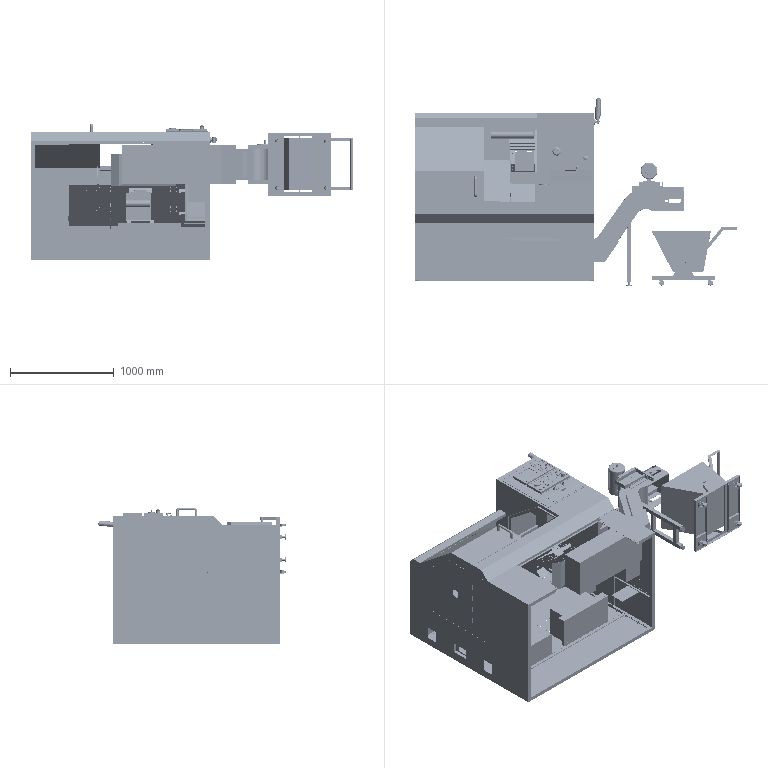Assembly | SolidWorks | mm | 112 component files | 213 solids | 6594 faces | box 3103.3 x 1799.75 x 1316.5 mm | volume 83821011 mm3 | plane 4108 | cylinder 2360 | cone 62 | torus 44 | sphere 16 | spline 4 | commonest cylinder face diameters 3 x356 4 x356 7 x259 6 x244 10 x225 5.2 x144 14 x52 8 x48
Bill of materials:
GuardWheel | 4 |  | L-shaped (right-angle) plate body carrying a long cylinder and a shorter cylinder, with slotted fork-like flat tabs at the cylinder ends.
Telescopic | 1 |  | Bent thin-sheet bracket with stepped/notched outline: a large flat panel, an offset narrower flange, and a downturned flange with an irregular notched edge.
Baffle | 1 |  | Thin flat U-shaped (inverted-U) plate with a large rectangular open cutout and many small through-holes, plus a downturned flange along one edge.
BaffleFixingBracket | 1 |  | Slender bent-strap bracket in a Z/offset shape, with U-channel style ends that each carry flat tabs with small holes.
Bracket | 2 |  | Long straight channel/angle strip formed as a folded right-angle (V-shaped) section, with two small holes along its length.
Cart | 1 |  | Open hopper/bin-like box with a trapezoidal (tapered) side profile, short pin stubs on opposite sides, and a bent rod-style handle loop sticking out of one side.
ChipCollectorCartChassis | 1 |  | Rectangular frame plate with a large central rectangular opening, side channel walls, and a tapered central tab ending in a small ring/eyelet.
TY-07-02-00BlackSmallRubberWheel | 4 |  | Caster-like wheel unit: square mounting plate with four corner holes, a fork/yoke bracket, and a single rounded cylindrical wheel on an axle.
Casing | 1 |  | Large sheet-metal style frame/enclosure with rectangular windows, a chamfered corner, folded side walls, and an attached long cantilever channel arm.
ChipConveyor1 | 1 |  | Elongated inclined channel/chute-like structure: a long box section that steps up through a curved incline to a raised head section with a plate and slots, held by a rod frame with a leg and knob-ended rods.
ControlBox | 1 |  | Shallow rectangular box/tray frame with a chamfered lower edge, two rectangular openings in the top, recessed side pockets, and round holes in the end walls.
ControlBoxDoor | 1 |  | Thin rectangular flat panel/lid with a rounded-corner rectangular slot (hand-hole like) and short pin stubs at both ends of one edge; a rolled or rounded lobe is seen along that edge.
ControlBoxRearPanel | 1 |  | Thin flat square plate with one small round through-hole near each of the four corners.
CopyOfSystem | 1 |  | Rectangular panel-style body made of a shallow top housing over a thin perimeter flange with mounting holes and a deeper, narrower rectangular box underneath. The top face has a raised rim border, a grid of small square key-like pads, a large round recess with a cylindrical boss inside it, a short pin, several low round buttons, a domed cylindrical knob, and a small rectangular block.
System | 1 |  | Rectangular housing with a flanged top. A thin perimeter flange with mounting holes sits on top of a deep rectangular box. The top surface is split into two raised sections: a larger one with a shallow rectangular recess and a row of small tabs along one edge, and a smaller one with a recessed field holding a grid of small square pads.
1_1 | 1 |  | Stepped cylindrical part: a larger-diameter head with a smaller-diameter shank below it. The head has a slot or partial cut-away, a cylindrical cross pin running through the slot, and the pin ends stick out slightly on both sides of the head. The shank has a chamfered end.
2_1 | 1 |  | Round bar or tube bent into a U shape, with two parallel legs joined by a long straight span through rounded bends. Each leg end has a small cross hole.
3_1 | 1 |  | Hexagonal nut-shaped body with a central round bore and chamfered corners on both faces.
4_1 | 1 |  | Plain flat annular washer-shaped ring: a circular disk with a concentric central hole and uniform thickness.
5_1 | 1 |  | Stepped cylindrical part: a larger-diameter head with a smaller-diameter shank below it. The head has a slot or partial cut-away, a cylindrical cross pin running through the slot, and the pin ends stick out slightly on both sides of the head. The shank has a chamfered end.
6 | 1 |  | Hexagonal nut-shaped body with a central round bore and chamfered corners.
7_1 | 1 |  | Plain flat annular washer-shaped ring: a circular disk with a concentric central hole and uniform thickness.
ControlBoxGasket | 2 |  | Very thin flat annular ring (shim-like): a circular disk with a large concentric central hole.
ControllerRotatingShaft | 2 |  | Flanged sleeve: a thin-walled cylindrical tube with a thin flat circular flange at one end, and four evenly spaced round through-holes in the flange.
Door | 1 | Plain Carbon Steel | Sheet panel bent into a profile with three sections: horizontal, sloped, and vertical. A large rounded-rectangle window is cut through the sloped section, and the panel has small holes and slots.
DoorGlass | 1 |  | Thin flat rectangular plate set at an incline, with no visible holes or features.
ElectricalBoxCoverPlate | 1 |  | Long, narrow, flat rectangular strip with small holes at both ends and at mid-length.
ElectricalBoxCoverPlate2 | 1 |  | Flat rectangular strip, shorter and wider in proportion than a long bar, with six small holes: four at the corners and two at mid-length.
FixedBracket2 | 1 |  | Bent sheet bracket with an L-shaped (angle) cross-section. One leg tapers along its length, and the other leg has two round holes.
FixedFrame | 1 |  | Bent sheet angle bracket similar to a tapered L-bracket, with two round holes in one leg and a tapered opposite leg; it appears to be mirrored or oriented differently from the similar part.
FrontBaffle | 1 |  | Sheet panel bent into a horizontal, sloped, and vertical section profile, with no large window, and with a row of small holes along the bent edges.
FrontReceivingPlate | 1 |  | Long bent angle strip with two legs at a non-right (acute) angle and tapered or angled cut ends.
FuelTank | 1 |  | Rectangular box-shaped body with a flange plate at one face that extends slightly beyond the box outline, with four corner holes. One hole is also visible on the top face.
FuelTankCap | 1 |  | Flat thin rectangular plate with four round holes near the corners.
1 | 1 |  | Complex multi-bend sheet bracket with several panels, side legs, notches, stepped tabs, and an offset cutout region.
2 | 1 |  | Bent sheet part with a broad, channel-like body, two side legs, a central opening between two sloped panels, and a small central tab with a hole.
3 | 1 |  | Thin bent sheet-metal panel: a large flat plate with a wide rectangular cutout that leaves two parallel legs, plus a narrow bent strip/flange along the solid edge carrying small holes; the side view shows the main plate inclined at roughly 45 degrees and a short stepped (Z-like) flange at one end.
TieRod1 | 4 |  | Flat bar link with fully rounded ends and one round through-hole near each end.
TieRod2 | 2 |  | Long, slender flat bar with rounded ends and three small through-holes, one at each end and one at mid-length.
GlassPressFrame | 1 |  | Thin flat rectangular frame or gasket-like plate with a large central rectangular opening and eight small holes around the border (four corners and four edge midpoints).
Handle | 1 |  | U-shaped bent round rod: one straight crossbar joined to two parallel straight legs by radiused bends, with the legs ending in flat cut faces.
IlluminationLamp | 1 |  | Elongated half-round (D-section) body with a flat back face and a curved front, closed at each end by a plate that projects past the flat side and has two small notches on its edge.
LampHolder | 1 |  | Sheet-metal hat-section channel: a web, two parallel side walls and outward-turned flanges along both free edges, with two small holes near each end of the web.
Base | 1 |  | Flanged bushing-like part: a circular flange disc with three through-holes, and a short, slightly tapered cylindrical hub with a central through-bore.
LED | 1 |  | Elongated cylindrical housing with a rounded closed end. The other end has a smaller stepped spigot with a bore, surrounded by a ring of small holes/pockets on the end face. There is a circular patch of parallel slots on the side near the spigot end, and faint circumferential seam lines along the body.
RotatingHead | 1 |  | Cylindrical disc/eye body with a central through-hole, plus a two-diameter stepped cylindrical pin projecting radially from its side; the underside face shows a small hole and an arc-shaped groove.
UpperRotatingHead | 1 |  | Cylindrical disc/eye body with a chamfered central through-bore, plus a two-diameter stepped cylindrical pin projecting radially from its side; the outer edges and pin end are chamfered.
LeftGuardBracket | 2 |  | Long sheet-metal angle bracket: an L-section strip with two round holes in one leg, plus a perpendicular bent end tab with a single round hole.
LeftLowerSkirt | 1 |  | L-shaped bent sheet: a long rectangular leg and a shorter perpendicular leg joined at one bend.
LeftMaterialInletPlate | 1 |  | Thin plate with a single obtuse bend, giving two flat panels at an angle.
LeftSideGuardPlate | 1 |  | Thin flat rectangular strip or plate with no visible holes.
LeftWindow | 1 |  | Flat panel with one chamfered (angled) corner, a large round hole, a grid of parallel slots, and small holes around the edge.
LowerBaffle | 1 |  | Thin flat plate with a stepped, chamfered upper outline and a rounded notch at one lower corner.
LowerRightPlateBracket | 1 |  | L-shaped bracket: a wide flat flange and a short perpendicular flange, each with two round holes.
LowerRightSurroundCoverPlate | 1 |  | Thin flat rectangular plate with one small round hole near each of the four corners.
MiddleBaffle | 1 |  | Flat polygonal plate with angled edges and stepped tabs, a large central circular opening, and many small holes.
Motor | 1 |  | Cylindrical body with lengthwise ribs, a small protruding shaft on one end, a rounded dome on the other end, a rectangular box on one side, and a flat foot base.
OilTankBracket | 1 |  | Wedge-shaped (tapered) solid block with small holes on two faces.
Axis | 2 |  | Flanged cylindrical bushing with a through-bore and a shallow ring-shaped groove near the top end.
Bearing | 2 |  | Short annular ring (washer- or bearing-like shape) with a central bore and concentric ring grooves on one face.
Pulley | 2 |  | Short ring with a through-bore and a groove around the outside, which gives it a spool-like profile of two thin outer flanges joined by a smaller-diameter hub.
RearBaffle | 1 |  | Thin rectangular plate with a low raised rim around its edge, like a shallow tray. It has twelve groups of short parallel slots and small pins or holes along two opposite edges.
RearCoverPlate | 1 |  | Long, shallow, open-faced rectangular pan or channel: a flat web with walls on all four edges. The walls have small holes.
RearFixingPlate | 1 |  | Thin, flat rectangular plate with four round through-holes in a rectangular pattern near the corners.
RearLowerSkirt | 1 |  | Long angle-shaped piece: a long flat base with a short upright wall at one end. It has a few small holes and a fine line or groove along one long edge.
RightSideBaffle | 1 |  | Rectangular block or bar with a step (notch) at one end. It is set at an angle to the view axes.
RightSideLowerBaffle | 1 |  | Bent sheet-metal panel: a tall flat main panel with a large stepped rectangular window cut out, and a 90-degree flange along the top. The flange has slotted holes and a stepped (notched) outline.
RightSideWindow | 1 |  | Very thin flat plate shaped like a five-sided polygon: a near-square with one corner cut off at about 45 degrees. It has small holes near the edges.
Telescopic1 | 1 |  | Bent sheet-metal bracket. In profile it has a sloped leg at about 45 degrees running into a horizontal leg that ends in a short turned-down lip. The sloped leg has stepped tabs, and the plan view shows a rectangular notch cut from one side.
Telescopic2 | 1 |  | Bent sheet-metal bracket with a profile similar to the previous bracket: a sloped leg into a horizontal leg ending in a short lip, with stepped tabs on the sloped leg. The plan view is a plain rectangle with no notch.
Telescopic3 | 1 |  | Bent bracket with a sloped leg joined to a horizontal leg. The sloped leg has two raised strips or tabs, each carrying a pair of small holes.
WheelAssembly | 4 |  | Compact L-shaped (90-degree) body with rectangular pockets that hold two cylinders of different lengths. Both cylinders have axial holes. There are forked (slotted) end tabs.
RoundBaffle | 1 |  | Thin flat ring (annulus) with four small through-holes spaced evenly around the rim.
ScraperPlate | 1 |  | Thin flat strip in a joggled/Z shape in plan: a straight end section, a diagonal middle section and a second straight end section, with a single row of small holes along the centerline.
Section1 | 1 |  | Formed sheet-metal channel or cover: a rectangular main panel with folded side walls, end walls with a stepped central notch along the bottom edge, and a small tab with a hole at one corner.
Section2 | 1 |  | Formed sheet-metal channel or cover: a rectangular panel with folded side and end walls, and end walls with a stepped notch along the bottom edge that has angled corners. Very similar to the other channel parts, but it has no corner tab hole.
Section3 | 1 |  | Formed sheet-metal channel or cover with folded walls and a stepped bottom-edge notch in the end walls. Its proportions are a little longer and narrower than the other channel variants.
Section4 | 1 |  | Formed sheet-metal channel or cover, the narrowest and most elongated of the similar variants, with folded walls and a stepped notch along the bottom edge in the end walls.
Section5 | 1 |  | Formed sheet-metal bracket: a central channel section with rectangular openings, and two angled mounting legs that each carry four elongated slots and have rounded corners.
SlideRail | 1 |  | Long, thin, flat bar with four evenly spaced small holes along its centerline.
ElectricalBoxDoor | 1 |  | Thin flat rectangular plate with one small elongated slot near one long edge. The slot has narrow extensions at each end.
ElectricalBoxTopPlate | 1 |  | Thin flat rectangular plate with one small round hole near each of its four corners.
TransformerBox | 1 |  | Rectangular box-shaped sheet-metal enclosure. It has small holes along its edges, two small rectangular cutouts in one long side wall, a rectangular patch or recess on the top face, and inturned flanges or a lip around one open or edge side.
TransformerBoxPlate | 1 |  | Flat rectangular plate with a large central rectangular opening and four round holes near the corners.
UpperSlideBearing | 2 |  | Short annular ring (thick washer/ring shape) with a central through-bore; one face shows concentric inner and outer rings separated by a recessed annular groove.
UpperSlideFixedBlock | 2 |  | Solid stepped cylinder: a large-diameter disc-like section with a smaller coaxial cylindrical boss projecting from one face.
UpperBaffle | 1 |  | Long straight prismatic profile of constant cross-section; the section is a bent bar with a short flat leg, an angled transition segment, and a longer perpendicular leg (a joggled/offset angle shape).
UpperCoverBracket2 | 1 |  | Thin-walled sheet-style bracket: two triangular side plates, each with a tapered lightening cutout with rounded corners, joined by a rectangular web with a large central opening and bent flanges carrying round holes.
UpperGuardBracket | 1 |  | Thin-walled sheet-style bracket similar to a U-shaped frame: two triangular side plates with large tapered rounded-corner lightening cutouts, joined by a crossbar, with leg flanges carrying elongated slots and round holes.
WaterPump | 1 |  | Compound cylindrical assembly-like body: a large cylinder with a rectangular block underneath, a thin square flange plate with four corner holes, and parallel rods plus a flat bar extending to a cylindrical end disc.
Mates:
1. coincident | Casing-1 face at (-858.301, 497.073, 511.481) dir (0, 0, 1) | Door-1 face at (-869.55, -18.434, 511.481) dir (0, 0, 1)
2. distance | Door-1 face at (-869.55, -314.434, 481.481) dir (0, -1, 0) | Casing-1 face at (-869.55, -318.434, 129.481) dir (0, 1, 0)
3. coincident | Casing-1 face at (-871.55, -30.485, 476.481) dir (0, 0, -1) | FrontBaffle-1 face at (-294.55, -318.432, 476.481) dir (0, 0, 1)
4. coincident | Casing-1 face at (-871.55, 371.566, 162.364) dir (0, -1, 0) | FrontBaffle-1 face at (-294.55, 371.566, 162.363) dir (0, 1, 0)
5. distance | FrontBaffle-1 face at (-294.55, -36.686, 386.009) dir (1, 0, 0) | Casing-1 face at (-869.55, 406.571, 129.481) dir (1, 0, 0)
6. coincident | Casing-1 face at (240.45, 497.073, -448.519) dir (-1, 0, 0) | UpperBaffle-1 face at (240.45, 486.18, 119.594) dir (1, 0, 0)
7. coincident | Casing-1 face at (-934.55, 541.566, 511.481) dir (0, 1, 0) | UpperBaffle-1 face at (240.45, 541.566, 136.486) dir (0, 1, 0)
8. concentric | Door-1 face at (-354.55, -345.434, 473.481) dir (0, 0, 1) r 3.5 | PulleyAssembly-1/Axis-1 face at (-354.55, -345.434, 482.181) dir (0, 0, 1) r 1.65
9. coincident | Door-1 face at (-269.55, -538.432, 483.481) dir (0, 0, 1) | PulleyAssembly-1/Axis-1 face at (-354.55, -345.434, 483.481) dir (0, 0, -1)
10. concentric | Door-1 face at (-754.55, -345.434, 473.481) dir (0, 0, 1) r 3.5 | PulleyAssembly-2/Axis-1 face at (-754.55, -345.434, 482.181) dir (0, 0, 1) r 1.65
11. coincident | Door-1 face at (-269.55, -538.432, 483.481) dir (0, 0, 1) | PulleyAssembly-2/Axis-1 face at (-754.55, -345.434, 483.481) dir (0, 0, -1)
12. coincident | Casing-1 face at (-858.301, 497.073, 491.481) dir (0, 0, -1) | SlideRail-1 face at (-791.2, -396.75, 491.481) dir (0, 0, 1)
13. distance | SlideRail-1 face at (235.45, -361.434, 491.481) dir (1, 0, 0) | Casing-1 face at (240.45, 497.073, -448.519) dir (-1, 0, 0)
14. tangent | PulleyAssembly-1/Pulley-1 face at (-354.55, -345.434, 494.431) dir (0, 0, 1) r 16 | SlideRail-1 face at (-897.55, -361.434, 491.481) dir (0, 1, 0)
15. tangent | PulleyAssembly-2/Pulley-1 face at (-754.55, -345.434, 494.431) dir (0, 0, 1) r 16 | SlideRail-1 face at (-897.55, -361.434, 491.481) dir (0, 1, 0)
16. coincident | Door-1 face at (-911.609, 394.568, -8.567) dir (0, -1, 0) | UpperAxis-1/UpperSlideFixedBlock-1 face at (-778.65, 394.568, -31.569) dir (0, 1, 0)
17. tangent | Door-1 face at (-776.05, 386.568, -35.567) dir (-1, 0, 0) | UpperAxis-1/UpperSlideFixedBlock-1 face at (-778.65, 386.568, -31.569) dir (0, 1, 0) r 2.6
18. tangent | Casing-1 face at (-858.301, 497.073, -17.569) dir (0, 0, -1) | UpperAxis-1/UpperSlideBearing-1 face at (-778.65, 382.968, -31.569) dir (0, 1, 0) r 14
19. coincident | Door-1 face at (-911.609, 394.568, -8.567) dir (0, -1, 0) | UpperAxis-2/UpperSlideFixedBlock-1 face at (-323.45, 394.568, -31.569) dir (0, 1, 0)
20. tangent | Door-1 face at (-326.05, 386.568, -35.567) dir (-1, 0, 0) | UpperAxis-2/UpperSlideFixedBlock-1 face at (-323.45, 386.568, -31.569) dir (0, 1, 0) r 2.6
21. tangent | Casing-1 face at (-858.301, 497.073, -17.569) dir (0, 0, -1) | UpperAxis-2/UpperSlideBearing-1 face at (-323.45, 382.968, -31.569) dir (0, 1, 0) r 14
22. coincident | Casing-1 face at (-858.301, 497.073, -448.519) dir (0, 0, -1) | TransformerBoxAssembly-1/TransformerBox-1 face at (-325.887, 480.248, -448.519) dir (0, 0, 1)
23. coincident | Casing-1 face at (-934.55, 541.566, 511.481) dir (0, 1, 0) | TransformerBoxAssembly-1/TransformerBox-1 face at (-249.55, 541.566, -723.519) dir (0, 1, 0)
24. coincident | Casing-1 face at (-934.55, 541.566, 511.481) dir (-1, 0, 0) | TransformerBoxAssembly-1/TransformerBox-1 face at (-934.55, 541.566, -723.519) dir (-1, 0, 0)
25. coincident | Casing-1 face at (-858.301, 497.073, -48.569) dir (0, 0, 1) | UpperBaffle-1 face at (240.45, 541.566, -48.569) dir (0, 0, -1)
26. distance | ControlAssembly-1/ControlBox-1 face at (265.455, 494.566, 511.485) dir (0, 1, 0) | Casing-1 face at (260.45, 496.566, 356.481) dir (0, -1, 0)
27. concentric | Casing-1 face at (310.45, 499.566, 461.481) dir (0, 1, 0) r 30 | ControlAssembly-1/ControlBox-1 face at (310.45, -230.286, 461.481) dir (0, 1, 0) r 30
28. coincident | Casing-1 face at (783.45, 497.073, -448.519) dir (1, 0, 0) | RightSideWindow-1 face at (783.45, 328.531, 142.879) dir (-1, 0, 0)
29. distance | RightSideWindow-1 face at (785.45, -137.434, 245.481) dir (0, 0, 1) | Casing-1 face at (775.45, -138.434, 246.481) dir (0, 0, -1)
30. distance | RightSideWindow-1 face at (785.45, 450.566, 191.456) dir (0, 1, 0) | Casing-1 face at (775.45, 451.566, 82.456) dir (0, -1, 0)
31. coincident | Casing-1 face at (-932.55, 497.073, -448.519) dir (-1, 0, 0) | LeftWindow-1 face at (-932.55, 184.645, 221.914) dir (1, 0, 0)
32. distance | LeftWindow-1 face at (-934.55, 230.566, -304.543) dir (0, 1, 0) | Casing-1 face at (-932.55, 231.566, 233.673) dir (0, -1, 0)
33. distance | LeftWindow-1 face at (-934.55, 3.986, 410.481) dir (0, 0, 1) | Casing-1 face at (-932.55, -518.434, 411.481) dir (0, 0, -1)
34. coincident | Casing-1 face at (785.45, 541.566, 511.481) dir (1, 0, 0) | RightSideLowerBaffle-1 face at (785.45, -518.434, 418.481) dir (1, 0, 0)
35. coincident | Casing-1 face at (-934.55, -518.434, 511.481) dir (0, -1, 0) | RightSideLowerBaffle-1 face at (748.616, -518.434, 359.008) dir (0, 1, 0)
36. coincident | RearBaffle-1 face at (624.236, -611.046, -723.519) dir (0, 0, -1) | RearLowerSkirt-1 face at (747.45, -698.434, -723.519) dir (0, 0, -1)
37. coincident | RightSideLowerBaffle-1 face at (747.45, -518.434, 418.481) dir (-1, 0, 0) | RearLowerSkirt-1 face at (747.45, -698.434, -723.519) dir (1, 0, 0)
38. coincident | TransformerBoxAssembly-1/TransformerBox-1 face at (-249.55, -698.434, -723.519) dir (0, -1, 0) | RearLowerSkirt-1 face at (-883.512, -698.434, -670.865) dir (0, 1, 0)
39. coincident | RearLowerSkirt-1 face at (-896.55, -698.434, -448.519) dir (0, 0, 1) | LeftLowerSkirt-1 face at (-934.55, -1068.434, -448.519) dir (0, 0, -1)
40. coincident | RearLowerSkirt-1 face at (-934.55, -698.434, -723.519) dir (-1, 0, 0) | LeftLowerSkirt-1 face at (-934.55, -1068.434, -448.519) dir (-1, 0, 0)
41. coincident | Casing-1 face at (-934.55, -518.434, 511.481) dir (0, -1, 0) | LeftLowerSkirt-1 face at (-869.411, -518.434, 355.553) dir (0, 1, 0)
42. coincident | ChipConveyor1-1 face at (1429.605, -126.434, 388.481) dir (0, 1, 0) | Motor-1 face at (1319.605, -126.434, 113.481) dir (0, -1, 0)
43. distance | Motor-1 face at (1379.605, -126.434, 178.481) dir (1, 0, 0) | ChipConveyor1-1 face at (1429.605, -126.434, 8.481) dir (1, 0, 0)
44. distance | ChipConveyor1-1 face at (1429.605, -126.434, 388.481) dir (0, 0, 1) | Motor-1 face at (1379.605, -126.434, 328.481) dir (0, 0, 1)
45. distance | RightTelescopicGuard-1/Telescopic3-1 face at (763.45, 118.931, 47.795) dir (1, 0, 0) | Casing-1 face at (783.45, 541.566, 511.481) dir (-1, 0, 0)
46. coincident | UpperGuardBracket-1 face at (42.462, 49.671, -350.102) dir (0, 0.7071, 0.7071) | UpperCoverBracket2-1 face at (-11.175, 329.475, -629.906) dir (0, -0.7071, -0.7071)
47. coincident | UpperGuardBracket-1 face at (248.825, 18.068, -381.705) dir (1, 0, 0) | UpperCoverBracket2-1 face at (248.825, 362.351, -588.779) dir (1, 0, 0)
48. concentric | UpperGuardBracket-1 face at (229.825, 205.235, -505.666) dir (0, -0.7071, -0.7071) r 5 | UpperCoverBracket2-1 face at (229.825, 206.649, -504.251) dir (0, -0.7071, -0.7071) r 5
49. concentric | UpperGuardBracket-1 face at (7.825, 148.666, -449.097) dir (0, -0.7071, -0.7071) r 5 | UpperCoverBracket2-1 face at (7.825, 150.08, -447.683) dir (0, -0.7071, -0.7071) r 5
50. coincident | GeneralAssembly-1/3-1 face at (24.377, 419.724, -539.658) dir (0, 0.7071, -0.7071) | UpperCoverBracket2-1 face at (-11.175, 434.834, -524.548) dir (0, -0.7071, 0.7071)
51. coincident | RightTelescopicGuard-1/Telescopic1-1 face at (588.825, 91.39, -391.236) dir (0, 0, 1) | Assembly-1/Telescopic-1 face at (-16.175, 91.39, -391.236) dir (0, 0, 1)
52. coincident | FixedFrame-1 face at (660.45, -211.958, -227.065) dir (0, 0.7071, 0.7071) | Bracket-1 face at (488.45, -199.938, -239.086) dir (0, -0.7071, -0.7071)
53. coincident | FixedBracket2-1 face at (660.45, -393.685, -45.339) dir (0, 0.7071, 0.7071) | Bracket-2 face at (488.45, -393.685, -45.339) dir (0, -0.7071, -0.7071)
54. coincident | RightTelescopicGuard-1/Telescopic1-1 face at (588.825, 91.39, -391.236) dir (0, 0, 1) | Baffle-1 face at (-6.409, 353.688, -391.236) dir (0, 0, -1)
55. distance | GeneralAssembly-1/3-1 face at (-30.175, 180.983, -450.301) dir (-1, 0, 0) | Baffle-1 face at (-35.175, 308.593, -391.236) dir (1, 0, 0)
56. distance | Baffle-1 face at (390.825, 308.593, -391.236) dir (0, -0.7071, -0.7071) | GeneralAssembly-1/3-1 face at (-30.175, 270.786, -360.499) dir (0, 0.7071, 0.7071)
57. coincident | Assembly-1/Telescopic-1 face at (-16.175, 91.39, -393.236) dir (0, 0, -1) | RearFixingPlate-1 face at (218.065, 400.589, -393.236) dir (0, 0, 1)
58. coincident | Assembly-1/Telescopic-1 face at (-16.175, 513.39, -393.236) dir (0, 1, 0) | RearFixingPlate-1 face at (147.825, 513.39, -393.236) dir (0, 1, 0)
59. distance | RightTelescopicGuard-1/Telescopic1-1 face at (407.825, 423.717, -411.168) dir (-1, 0, 0) | RearFixingPlate-1 face at (347.825, 513.39, -393.236) dir (1, 0, 0)
60. coincident | GeneralAssembly-1/1-1 face at (341.825, 228.737, -335.421) dir (1, 0, 0) | RightSideBaffle-1 face at (341.825, -170.778, 64.094) dir (1, 0, 0)
61. coincident | GeneralAssembly-1/1-1 face at (28.168, 169.698, -295.465) dir (0, -0.7071, 0.7071) | LeftSideGuardPlate-1 face at (-18.175, 177.826, -287.338) dir (0, 0.7071, -0.7071)
62. coincident | Casing-1 face at (-299.55, -318.434, 476.48) dir (0, 0, 1) | LowerBaffle-2 face at (-297.55, -378.434, 476.48) dir (0, 0, 1)
63. coincident | FrontBaffle-1 face at (-294.55, -36.686, 386.009) dir (1, 0, 0) | MiddleBaffle-1 face at (-294.55, -248.256, 346.681) dir (-1, 0, 0)
64. concentric | FrontBaffle-1 face at (-296.55, -268.432, 461.481) dir (1, 0, 0) r 3 | MiddleBaffle-1 face at (-292.55, -268.432, 461.481) dir (-1, 0, 0) r 3
65. concentric | FrontBaffle-1 face at (-296.55, -53.432, 461.481) dir (1, 0, 0) r 3 | MiddleBaffle-1 face at (-292.55, -53.432, 461.481) dir (-1, 0, 0) r 3
66. coincident | MiddleBaffle-1 face at (-292.55, -248.256, 346.681) dir (1, 0, 0) | RoundBaffle-1 face at (-292.55, -77.904, 57.481) dir (-1, 0, 0)
67. coincident | MiddleBaffle-1 face at (-292.55, -248.256, 346.681) dir (1, 0, 0) | ScraperPlate-1 face at (-292.55, -121.313, -21.856) dir (-1, 0, 0)
68. distance | ScraperPlate-1 face at (-279.55, 368.876, -387.236) dir (0, 0, -1) | Assembly-1/Telescopic-1 face at (-16.175, 91.39, -391.236) dir (0, 0, 1)
69. distance | Assembly-1/Telescopic-1 face at (-16.175, -359.744, 60.727) dir (0, 0.7071, 0.7071) | ScraperPlate-1 edge at (-279.55, 93.876, -387.236) dir (0, -0.7071, 0.7071)
70. coincident | MiddleBaffle-1 face at (-319.55, -248.256, 346.681) dir (-1, 0, 0) | BaffleFixingBracket-1 face at (-319.55, 159.566, -298.231) dir (1, 0, 0)
71. coincident | Casing-1 face at (-775.795, 519.566, -356.519) dir (0, -1, 0) | BaffleFixingBracket-1 face at (-571.279, 519.566, -298.231) dir (0, 1, 0)
72. distance | BaffleFixingBracket-1 face at (-439.962, 464.133, -298.231) dir (0, 0, 1) | MiddleBaffle-1 face at (-319.55, 288.552, -303.231) dir (0, 0, 1)
73. coincident | Casing-1 face at (-858.301, 539.566, -448.519) dir (0, 1, 0) | ElectricalBoxCoverPlate2-1 face at (311.826, 539.566, 414.962) dir (0, -1, 0)
74. distance | ElectricalBoxCoverPlate2-1 face at (276.45, 541.566, 490.481) dir (-1, 0, 0) | Casing-1 face at (275.45, 539.566, -133.519) dir (1, 0, 0)
75. distance | ElectricalBoxCoverPlate2-1 face at (276.45, 541.566, 490.481) dir (0, 0, 1) | Casing-1 face at (365.45, 539.566, 491.481) dir (0, 0, -1)
76. coincident | Casing-1 face at (-858.301, 497.073, -448.519) dir (0, 0, -1) | RearCoverPlate-1 face at (744.45, 541.566, -448.519) dir (0, 0, 1)
77. coincident | Casing-1 face at (-934.55, 541.566, 511.481) dir (0, 1, 0) | RearCoverPlate-1 face at (671.234, 541.566, -640.192) dir (0, 1, 0)
78. distance | RearCoverPlate-1 face at (744.45, 541.566, -448.519) dir (1, 0, 0) | Casing-1 face at (745.45, -516.434, -345.519) dir (-1, 0, 0)
79. distance | Casing-1 face at (745.45, -516.434, -345.519) dir (-1, 0, 0) | RearBaffle-1 face at (744.45, 541.566, -723.519) dir (1, 0, 0)
80. distance | LowerRightPlateBracket-1 face at (763.45, -726.416, -398.519) dir (1, 0, 0) | RightSideLowerBaffle-1 face at (783.45, -518.434, 418.481) dir (-1, 0, 0)
81. distance | Casing-1 face at (-869.55, 406.571, 129.481) dir (1, 0, 0) | Door-1 face at (-869.55, -538.432, 521.433) dir (-1, 0, 0)
82. coincident | Casing-1 face at (-858.301, 539.566, -448.519) dir (0, 1, 0) | ElectricalBoxCoverPlate-1 face at (-747.877, 539.566, -196.261) dir (0, -1, 0)
83. distance | Casing-1 face at (-814.55, 539.566, -223.519) dir (1, 0, 0) | ElectricalBoxCoverPlate-1 face at (-813.55, 541.566, -222.519) dir (-1, 0, 0)
84. distance | ElectricalBoxCoverPlate-1 face at (-813.55, 541.566, -134.519) dir (0, 0, 1) | Casing-1 face at (-814.55, 539.566, -133.519) dir (0, 0, -1)
85. coincident | RightSideLowerBaffle-1 face at (783.45, -1068.434, 359.008) dir (1, 0, 0) | LowerRightSurroundCoverPlate-1 face at (783.45, -853.152, -210.712) dir (-1, 0, 0)
86. distance | LowerRightSurroundCoverPlate-1 face at (785.45, -589.434, 1.481) dir (0, 1, 0) | RightSideLowerBaffle-1 face at (793.45, -588.434, -248.519) dir (0, -1, 0)
87. distance | RightSideLowerBaffle-1 face at (793.45, -588.434, -248.519) dir (0, 0, 1) | LowerRightSurroundCoverPlate-1 face at (785.45, -589.434, -247.519) dir (0, 0, -1)
88. distance | Section2-1 face at (-10.175, -359.222, 100.51) dir (-1, 0, 0) | Section1-1 face at (-14.175, -274.723, 12.476) dir (1, 0, 0)
89. distance | Section2-1 face at (-10.175, -317.149, 142.583) dir (0, 0.7071, 0.7071) | Section1-1 face at (-16.175, -228.054, 59.145) dir (0, -0.7071, -0.7071)
90. distance | Section1-1 face at (41.324, -231.589, 55.609) dir (0, -0.7071, 0.7071) | Section2-1 face at (47.324, -322.099, 137.633) dir (0, -0.7071, 0.7071)
91. distance | Section3-1 face at (-4.175, -443.721, 188.545) dir (-1, 0, 0) | Section2-1 face at (-8.175, -359.222, 100.51) dir (1, 0, 0)
92. distance | Section3-1 face at (-4.175, -407.659, 224.608) dir (0, 0.7071, 0.7071) | Section2-1 face at (-10.175, -318.563, 141.169) dir (0, -0.7071, -0.7071)
93. distance | Section2-1 face at (47.324, -322.099, 137.633) dir (0, -0.7071, 0.7071) | Section3-1 face at (53.324, -412.609, 219.658) dir (0, -0.7071, 0.7071)
94. distance | Section3-1 face at (-4.175, -409.073, 223.193) dir (0, -0.7071, -0.7071) | Section4-1 face at (1.825, -425.79, 234.254) dir (0, 0.7071, 0.7071)
95. distance | Section4-1 face at (1.825, -455.842, 204.202) dir (-1, 0, 0) | Section3-1 face at (-2.175, -443.721, 188.545) dir (1, 0, 0)
96. distance | Section4-1 face at (-2140.123, -434.908, 225.136) dir (0, -0.7071, 0.7071) | Section3-1 face at (53.324, -412.609, 219.658) dir (0, -0.7071, 0.7071)
97. distance | Section5-1 face at (7.825, -466.802, 266.781) dir (0, 0.7071, 0.7071) | Section4-1 face at (1.825, -427.204, 232.839) dir (0, -0.7071, -0.7071)
98. distance | Section5-1 face at (7.825, -490.844, 242.739) dir (-1, 0, 0) | Section4-1 face at (3.825, -455.842, 204.202) dir (1, 0, 0)
99. distance | Section4-1 face at (-2140.123, -434.908, 225.136) dir (0, -0.7071, 0.7071) | Section5-1 face at (69.561, -482.545, 253.866) dir (0, -0.7071, 0.7071)
100. coincident | ChipConveyor1-1 face at (908.45, -696.434, 198.481) dir (0, 1, 0) | WaterPump-1 face at (820.708, -696.434, -162.183) dir (0, -1, 0)
101. coincident | ChipConveyor1-1 edge at (671.45, -698.434, -73.519) dir (0, 1, 0) r 50 | WaterPump-1 face at (671.45, -551.434, -73.519) dir (0, -1, 0) r 50
102. concentric | ChipConveyor1-1 face at (625.95, -698.434, -119.019) dir (0, 1, 0) r 2.6 | WaterPump-1 face at (625.95, -691.434, -119.019) dir (0, -1, 0) r 4.5
103. coincident | Door-1 face at (-869.55, 405.337, 177.857) dir (0, -0.6157, -0.788) | DoorGlass-1 face at (-657.232, 290.803, 267.341) dir (0, 0.6157, 0.788)
104. distance | DoorGlass-1 face at (-350.55, 318.392, 245.786) dir (1, 0, 0) | Door-1 face at (-349.55, 317.948, 243.594) dir (-1, 0, 0)
105. distance | DoorGlass-1 face at (-788.55, 52.044, 453.88) dir (0, -0.788, 0.6157) | Door-1 face at (-349.55, 50.025, 452.919) dir (0, 0.788, -0.6157)
106. coincident | Door-1 face at (-269.55, -348.623, 764.377) dir (0, -0.6157, -0.788) | GlassPressFrame-1 face at (-749.348, 311.867, 248.345) dir (0, 0.6157, 0.788)
107. coincident | Door-1 face at (-349.55, 333.709, 231.281) dir (0, 0.788, -0.6157) | GlassPressFrame-1 face at (-809.55, 333.709, 231.281) dir (0, 0.788, -0.6157)
108. coincident | Door-1 face at (-329.55, 317.948, 243.594) dir (1, 0, 0) | GlassPressFrame-1 face at (-329.55, 333.709, 231.281) dir (1, 0, 0)
109. concentric | Door-1 face at (-349.55, -76.849, 509.481) dir (0, 0, 1) r 5 | Handle-1 face at (-349.55, -76.849, 558.481) dir (0, 0, -1) r 12.5
110. concentric | Door-1 face at (-349.55, -256.849, 509.481) dir (0, 0, 1) r 5 | Handle-1 face at (-349.55, -256.849, 558.481) dir (0, 0, -1) r 12.5
111. coincident | Door-1 face at (-869.55, -18.434, 511.481) dir (0, 0, 1) | Handle-1 face at (-349.55, -76.849, 511.481) dir (0, 0, -1)
112. coincident | FuelTank-1/FuelTank-1 face at (-34.55, -708.434, -371.519) dir (0, -1, 0) | OilTankBracket-1 face at (-91.55, -708.434, -368.519) dir (0, 1, 0)
113. coincident | FuelTank-1/FuelTank-1 face at (31.852, -500.162, -371.519) dir (0, 0, 1) | OilTankBracket-1 face at (-91.55, -631.434, -371.519) dir (0, 0, -1)
114. distance | Cart-1/ChipCollectorCartChassis-1 face at (1950.978, -1031.434, -101.519) dir (1, 0, 0) | ChipConveyor1-1 face at (1146.492, -462.442, 68.481) dir (1, 0, 0)
115. distance | Cart-1/Cart-1 face at (1593.152, -961.792, 448.481) dir (0, 0, 1) | ChipConveyor1-1 face at (908.45, -851.434, 348.481) dir (0, 0, 1)
116. coincident | ControlAssembly-1/ControlBox-1 face at (785.455, 494.566, 511.434) dir (1, 0, -0.00009864) | LEDAlarm-1/Base-1 face at (785.448, 455.307, 436.341) dir (-1, 0, 0.00009864)
117. concentric | ControlAssembly-1/ControlBox-1 face at (783.447, 475.267, 431.684) dir (1, 0, -0.00009864) r 2.6 | LEDAlarm-1/Base-1 face at (815.447, 475.267, 431.681) dir (-1, 0, 0.00009864) r 3
118. concentric | ControlAssembly-1/ControlBox-1 face at (783.446, 441.294, 421.385) dir (1, 0, -0.00009864) r 2.6 | LEDAlarm-1/Base-1 face at (815.446, 441.294, 421.381) dir (-1, 0, 0.00009864) r 3
119. coincident | FrontReceivingPlate-1 face at (-48.973, -635.077, -11.519) dir (0, 0, 1) | LeftMaterialInletPlate-1 face at (-159.009, -619.287, -11.519) dir (0, 0, -1)
120. coincident | Casing-1 face at (-858.301, 497.566, -448.519) dir (0, -1, 0) | LampHolder-1 face at (255.45, 497.566, -141.519) dir (0, 1, 0)
121. coincident | Casing-1 face at (-824.55, 499.566, -121.519) dir (0, 0, 1) | LampHolder-1 face at (255.45, 495.566, -121.519) dir (0, 0, 1)
122. distance | LampHolder-1 face at (-244.55, 457.638, -183.034) dir (-1, 0, 0) | Casing-1 face at (-294.55, 497.073, -448.519) dir (1, 0, 0)
123. concentric | LampHolder-1 face at (218.95, 373.566, -162.519) dir (0, -1, 0) r 2.6 | IlluminationLamp-1 face at (218.95, 368.566, -162.519) dir (0, -1, 0) r 3.25
124. concentric | LampHolder-1 face at (218.95, 373.566, -194.519) dir (0, -1, 0) r 2.6 | IlluminationLamp-1 face at (218.95, 368.566, -194.519) dir (0, -1, 0) r 3.25
125. coincident | LampHolder-1 face at (255.45, 371.566, -215.519) dir (0, -1, 0) | IlluminationLamp-1 face at (209.45, 371.566, -143.519) dir (0, 1, 0)
126. coincident | RearCoverPlate-1 face at (671.234, 541.566, -640.192) dir (0, 1, 0) | RearBaffle-1 face at (744.45, 541.566, -723.519) dir (0, 1, 0)
127. coincident | ControlAssembly-1/ControlBox-1 face at (265.455, -143.434, 511.485) dir (0, 1, 0) | ControllerRotatingShaft-1 face at (310.45, -143.434, 461.481) dir (0, -1, 0)
128. concentric | Casing-1 face at (310.45, -235.286, 461.481) dir (0, 1, 0) r 30 | ControllerRotatingShaft-1 face at (310.45, -143.434, 461.481) dir (0, -1, 0) r 29
129. coincident | ControlAssembly-1/ControlBox-1 face at (265.455, 492.566, 511.485) dir (0, -1, 0) | ControllerRotatingShaft-2 face at (310.45, 492.566, 461.481) dir (0, 1, 0)
130. concentric | Casing-1 face at (310.45, 499.566, 461.481) dir (0, -1, 0) r 30 | ControllerRotatingShaft-2 face at (310.45, 492.566, 461.481) dir (0, 1, 0) r 29
131. coincident | Casing-1 face at (260.45, -148.434, 356.481) dir (0, 1, 0) | ControlBoxGasket-1 face at (310.45, -148.434, 461.481) dir (0, -1, 0)
132. concentric | ControllerRotatingShaft-1 face at (310.45, -143.434, 461.481) dir (0, -1, 0) r 29 | ControlBoxGasket-1 face at (310.45, -146.434, 461.481) dir (0, -1, 0) r 45
133. coincident | ControlAssembly-1/ControlBox-1 face at (265.455, 494.566, 511.485) dir (0, 1, 0) | ControlBoxGasket-2 face at (310.45, 494.566, 461.481) dir (0, -1, 0)
134. concentric | ControllerRotatingShaft-2 face at (310.45, 492.566, 461.481) dir (0, 1, 0) r 29 | ControlBoxGasket-2 face at (310.45, 496.566, 461.481) dir (0, -1, 0) r 30
135. coincident | Telescopic-1 face at (-231.437, -358.968, 32.463) dir (-0.7071, -0.7071, 0) | GuardWheel-4 face at (-231.437, -358.968, 30.463) dir (0.7071, 0.7071, 0)
136. coincident | Telescopic-1 face at (-277.396, -404.928, 32.463) dir (0.7071, -0.7071, 0) | GuardWheel-4 face at (-224.366, -351.897, 30.463) dir (-0.7071, 0.7071, 0)
137. coincident | Telescopic-1 face at (132.981, 401.867, 30.463) dir (0, 0, -1) | GuardWheel-4 face at (-224.366, -351.897, 30.463) dir (0, 0, 1)
138. coincident | Telescopic-1 face at (-231.437, -358.968, -71.537) dir (0.7071, -0.7071, 0) | GuardWheel-2 face at (-224.366, -351.897, -72.537) dir (-0.7071, 0.7071, 0)
139. coincident | Telescopic-1 face at (-210.224, -380.182, -71.537) dir (-0.7071, -0.7071, 0) | GuardWheel-2 face at (-231.437, -358.968, -72.537) dir (0.7071, 0.7071, 0)
140. coincident | Telescopic-1 face at (132.981, 401.867, -69.537) dir (0, 0, 1) | GuardWheel-2 face at (-224.366, -351.897, -69.537) dir (0, 0, -1)
141. coincident | Telescopic-1 face at (132.981, 401.867, 30.463) dir (0, 0, -1) | GuardWheel-3 face at (-30.618, -158.15, 30.463) dir (0, 0, 1)
142. coincident | Telescopic-1 face at (-235.898, 32.988, 32.463) dir (-0.7071, -0.7071, 0) | GuardWheel-3 face at (-37.69, -165.221, 30.463) dir (0.7071, 0.7071, 0)
143. coincident | Telescopic-1 face at (331.19, 203.658, 32.463) dir (0.7071, -0.7071, 0) | GuardWheel-3 edge at (-71.631, -199.162, 30.463) dir (0, 0, 1)
144. coincident | Telescopic-1 face at (-37.69, -165.221, -71.537) dir (0.7071, -0.7071, 0) | GuardWheel-1 face at (-30.618, -158.15, -71.537) dir (-0.7071, 0.7071, 0)
145. coincident | Telescopic-1 face at (-16.476, -186.434, -71.537) dir (-0.7071, -0.7071, 0) | GuardWheel-1 face at (-37.69, -165.221, -71.537) dir (0.7071, 0.7071, 0)
146. coincident | Telescopic-1 face at (132.981, 401.867, -71.537) dir (0, 0, -1) | GuardWheel-1 face at (-30.618, -158.15, -71.537) dir (0, 0, 1)
147. distance | ChipCollectorCartChassis-1 face at (-292.759, -254.057, -40.297) dir (0, 1, 0) | Cart-1 face at (-110.057, -234.057, 59.345) dir (0, -1, 0)
148. concentric | ChipCollectorCartChassis-1 face at (-52.231, -254.057, 129.703) dir (0, -1, 0) r 10 | Cart-1 face at (-52.231, -232.057, 129.703) dir (0, -1, 0) r 9
149. coincident | ChipCollectorCartChassis-1 face at (-292.759, 278.379, -32.297) dir (0, 0, -1) | TY-07-02-00BlackSmallRubberWheel-1 face at (-263.231, 273.943, -32.297) dir (0, 0, 1)
150. distance | TY-07-02-00BlackSmallRubberWheel-1 face at (-263.231, 273.943, -32.297) dir (0, 1, 0) | ChipCollectorCartChassis-1 face at (-352.231, 313.943, -10.297) dir (0, -1, 0)
151. distance | TY-07-02-00BlackSmallRubberWheel-1 face at (-310.231, 273.943, -32.297) dir (-1, 0, 0) | ChipCollectorCartChassis-1 face at (-350.231, 315.943, -10.297) dir (1, 0, 0)
152. coincident | ChipCollectorCartChassis-1 face at (-292.759, 278.379, -32.297) dir (0, 0, -1) | TY-07-02-00BlackSmallRubberWheel-2 face at (205.769, 273.943, -32.297) dir (0, 0, 1)
153. coincident | ChipCollectorCartChassis-1 face at (-292.759, 278.379, -32.297) dir (0, 0, -1) | TY-07-02-00BlackSmallRubberWheel-3 face at (-263.231, -182.057, -32.297) dir (0, 0, 1)
154. coincident | ChipCollectorCartChassis-1 face at (-292.759, 278.379, -32.297) dir (0, 0, -1) | TY-07-02-00BlackSmallRubberWheel-4 face at (205.769, -182.057, -32.297) dir (0, 0, 1)
155. distance | ChipCollectorCartChassis-1 face at (245.769, 315.943, -10.297) dir (-1, 0, 0) | TY-07-02-00BlackSmallRubberWheel-4 face at (205.769, -182.057, -32.297) dir (1, 0, 0)
156. distance | TY-07-02-00BlackSmallRubberWheel-4 face at (205.769, -242.057, -32.297) dir (0, -1, 0) | ChipCollectorCartChassis-1 face at (-352.231, -282.057, -10.297) dir (0, 1, 0)
157. distance | ChipCollectorCartChassis-1 face at (245.769, 315.943, -10.297) dir (-1, 0, 0) | TY-07-02-00BlackSmallRubberWheel-2 face at (205.769, 273.943, -32.297) dir (1, 0, 0)
158. distance | TY-07-02-00BlackSmallRubberWheel-2 face at (205.769, 273.943, -32.297) dir (0, 1, 0) | ChipCollectorCartChassis-1 face at (-352.231, 313.943, -10.297) dir (0, -1, 0)
159. distance | TY-07-02-00BlackSmallRubberWheel-3 face at (-263.231, -242.057, -32.297) dir (0, -1, 0) | ChipCollectorCartChassis-1 face at (-352.231, -282.057, -10.297) dir (0, 1, 0)
160. distance | ChipCollectorCartChassis-1 face at (-350.231, 315.943, -10.297) dir (1, 0, 0) | TY-07-02-00BlackSmallRubberWheel-3 face at (-310.231, -182.057, -32.297) dir (-1, 0, 0)
161. coincident | ControlBox-1 face at (-251.115, 219.884, 92.304) dir (0, 0, 1) | System-2 face at (-145.281, 184.15, 92.304) dir (0, 0, -1)
162. coincident | ControlBox-1 face at (-251.115, 219.884, 92.304) dir (0, 0, 1) | CopyOfSystem-2 face at (-145.281, -15.85, 92.304) dir (0, 0, -1)
163. distance | CopyOfSystem-2 face at (137.807, 13.554, 52.304) dir (0, 1, 0) | ControlBox-1 face at (172.484, 14.554, 90.304) dir (0, -1, 0)
164. distance | CopyOfSystem-2 face at (-217.516, 21.554, 95.304) dir (-1, 0, 0) | ControlBox-1 face at (-207.516, 14.554, 90.304) dir (1, 0, 0)
165. distance | System-2 face at (137.807, 213.554, -17.396) dir (0, 1, 0) | ControlBox-1 face at (172.484, 214.554, 90.304) dir (0, -1, 0)
166. distance | System-2 face at (182.484, 221.554, 95.304) dir (1, 0, 0) | ControlBox-1 face at (172.484, 214.554, 90.304) dir (-1, 0, 0)
167. coincident | ControlBox-1 face at (-251.115, 219.884, -55.696) dir (0, 0, -1) | ControlBoxRearPanel-1 face at (-170.925, 193.367, -55.696) dir (0, 0, 1)
168. distance | ControlBoxRearPanel-1 face at (-226.516, 221.554, -55.696) dir (0, 1, 0) | ControlBox-1 face at (162.484, 222.554, -55.696) dir (0, -1, 0)
169. distance | ControlBoxRearPanel-1 face at (161.484, 221.554, -55.696) dir (1, 0, 0) | ControlBox-1 face at (162.484, 222.554, -55.696) dir (-1, 0, 0)
170. distance | ControlBoxDoor-1 face at (-216.516, -242.445, 92.276) dir (-1, 0, 0) | ControlBox-1 face at (-217.516, -241.446, 82.304) dir (1, 0, 0)
171. concentric | ControlBox-1 face at (-322.87, -357.446, 87.304) dir (1, 0, 0) r 2.6 | ControlBoxDoor-1 face at (-224.516, -357.446, 87.304) dir (1, 0, 0) r 2.5
172. coincident | ControlBox-1 face at (-251.115, 219.884, 92.304) dir (0, 0, 1) | UWAFN120-1/1_1-1 face at (40.254, -211.446, 92.304) dir (0, 0, -1)
173. concentric | ControlBox-1 face at (-77.516, -211.446, 90.304) dir (0, 0, 1) r 3 | UWAFN120-1/5_1-1 face at (-77.516, -211.446, 102.304) dir (0, 0, -1) r 2.6
174. concentric | ControlBox-1 face at (42.484, -211.446, 90.304) dir (0, 0, 1) r 3 | UWAFN120-1/1_1-1 face at (42.484, -211.446, 99.574) dir (0, 0, -1) r 5
175. concentric | 1_1-1 face at (0, -6.729, 0) dir (0, -1, 0) r 5 | 4_1-1 face at (0, -2, 0) dir (0, 1, 0) r 5
176. coincident | 3_1-1 face at (0.9465, -3, -3.886) dir (0, 1, 0) | 4_1-1 face at (0, -3, -7) dir (0, -1, 0)
177. concentric | 5_1-1 face at (120, -6.729, 0) dir (0, -1, 0) r 5 | 7_1-1 face at (120, -2, 0) dir (0, 1, 0) r 5
178. coincident | 6-1 face at (116, -3, 0) dir (0, 1, 0) | 7_1-1 face at (120, -3, -7) dir (0, -1, 0)
179. coincident | 4_1-1 face at (0, -1, -7) dir (0, 1, 0) | 7_1-1 face at (120, -1, -7) dir (0, 1, 0)
180. concentric | 2_1-1 face at (125, 10, 0) dir (-1, 0, 0) r 1 | 5_1-1 face at (120, 10, 0) dir (1, 0, 0) r 1
181. coincident | 1_1-1 plane at (0, 0, 0) dir (1, 0, 0) | 2_1-1 plane at (0, 6.579, 9.397) dir (1, 0, 0)
182. angle | 2_1-1 plane at (0, 6.579, 9.397) dir (0, 0.9397, 0.3421) | 1_1-1 plane at (0, 0, 0) dir (0, 0, 1)
183. distance | 7_1-1 face at (120, -1, -7) dir (0, 1, 0) | 5_1-1 face at (124.5, 0, 0) dir (0, -1, 0)
184. concentric | 1_1-1 face at (0, -6.729, 0) dir (0, -1, 0) r 5 | 3_1-1 face at (0, -12.43, 0) dir (0, -1, 0) r 5.001
185. concentric | 5_1-1 face at (120, -6.729, 0) dir (0, -1, 0) r 5 | 6-1 face at (120, -12.43, 0) dir (0, -1, 0) r 5.001
186. coincident | FuelTank-1 face at (-176.597, 131.067, -162.421) dir (0, 1, 0) | FuelTankCap-1 face at (-174.42, 131.067, 102.215) dir (0, -1, 0)
187. distance | FuelTankCap-1 face at (-238.999, 131.067, 133.579) dir (0, 0, 1) | FuelTank-1 face at (-176.597, 102.339, 134.579) dir (0, 0, -1)
188. distance | FuelTankCap-1 face at (193.001, 131.067, 133.579) dir (1, 0, 0) | FuelTank-1 face at (194.001, 134.067, 137.579) dir (-1, 0, 0)
189. distance | 1-1 face at (-305.803, 60.58, 139.006) dir (0, 1, 0) | 2-1 face at (-311.803, 64.58, -94.106) dir (0, -1, 0)
190. distance | 1-1 face at (54.197, 60.58, 139.006) dir (1, 0, 0) | 2-1 face at (58.197, 66.58, -94.106) dir (-1, 0, 0)
191. distance | 2-1 face at (-311.803, 66.58, -94.106) dir (0, 1, 0) | 3-1 face at (-317.803, 70.58, -327.218) dir (0, -1, 0)
192. distance | 2-1 face at (60.197, 66.58, -94.106) dir (1, 0, 0) | 3-1 face at (64.197, 72.58, -327.218) dir (-1, 0, 0)
193. coincident | 3-1 face at (-263.251, 39.58, -557.218) dir (0, -1, 0) | TieRod1-1 face at (-147.207, 39.58, -455.79) dir (0, 1, 0)
194. concentric | 3-1 face at (-128.303, 41.58, -554.218) dir (0, -1, 0) r 3 | TieRod1-1 face at (-128.303, 40.58, -554.218) dir (0, -1, 0) r 3
195. coincident | TieRod1-1 face at (-147.207, 35.58, -455.79) dir (0, -1, 0) | TieRod1-2 face at (-128.393, 35.58, -531.589) dir (0, 1, 0)
196. concentric | TieRod1-1 face at (-128.303, 40.58, -554.218) dir (0, -1, 0) r 3 | TieRod1-2 face at (-128.303, 36.58, -554.218) dir (0, -1, 0) r 3
197. coincident | TieRod1-2 face at (-128.393, 35.58, -531.589) dir (0, 1, 0) | TieRod2-1 face at (-151.107, 35.58, -254.023) dir (0, -1, 0)
198. concentric | TieRod1-2 face at (-98.648, 36.58, -435.877) dir (0, -1, 0) r 3 | TieRod2-1 face at (-98.648, 40.58, -435.877) dir (0, -1, 0) r 3
199. coincident | TieRod1-1 face at (-147.207, 35.58, -455.79) dir (0, -1, 0) | TieRod2-2 face at (-118.462, 35.58, -250.775) dir (0, 1, 0)
200. concentric | TieRod1-1 face at (-157.958, 40.58, -435.877) dir (0, -1, 0) r 3 | TieRod2-2 face at (-157.958, 36.58, -435.877) dir (0, -1, 0) r 3
201. concentric | TieRod2-1 face at (-128.303, 40.58, -317.536) dir (0, -1, 0) r 3 | TieRod2-2 face at (-128.303, 36.58, -317.536) dir (0, -1, 0) r 3
202. concentric | 2-1 face at (-128.303, 41.58, -317.536) dir (0, -1, 0) r 3 | TieRod2-2 face at (-128.303, 36.58, -317.536) dir (0, -1, 0) r 3
203. coincident | TieRod2-1 face at (-151.107, 35.58, -254.023) dir (0, -1, 0) | TieRod1-5 face at (-139.053, 35.58, -100.767) dir (0, 1, 0)
204. concentric | TieRod2-1 face at (-157.958, 40.58, -199.195) dir (0, -1, 0) r 3 | TieRod1-5 face at (-157.958, 30.58, -199.195) dir (0, 1, 0) r 3
205. concentric | 1-1 face at (-128.303, 41.58, -80.854) dir (0, -1, 0) r 3 | TieRod1-5 face at (-128.303, 30.58, -80.854) dir (0, 1, 0) r 3
206. coincident | TieRod2-2 face at (-118.462, 35.58, -250.775) dir (0, 1, 0) | TieRod1-6 face at (-117.536, 35.58, -100.758) dir (0, -1, 0)
207. concentric | TieRod1-5 face at (-128.303, 30.58, -80.854) dir (0, 1, 0) r 3 | TieRod1-6 face at (-128.303, 40.58, -80.854) dir (0, -1, 0) r 3
208. distance | TieRod2-2 face at (-98.648, 36.58, -199.195) dir (0, -1, 0) r 3 | TieRod1-6 face at (-98.551, 40.58, -199.171) dir (0, -1, 0) r 3
209. concentric | Base-1 face at (-74.588, 15.5, 41.329) dir (0, 0, -1) r 9 | UpperRotatingHead-1 face at (-74.588, 15.5, 18.329) dir (0, 0, 1) r 5.75
210. tangent | Base-1 face at (-74.588, 15.5, 41.329) dir (0, 0, 1) | UpperRotatingHead-1 face at (-83.199, 12.883, 57.829) dir (0.9568, 0.2908, 0) r 16.5
211. concentric | RotatingHead-1 face at (-54.495, 21.606, 57.829) dir (-0.9568, -0.2908, 0) r 5 | UpperRotatingHead-1 face at (-83.199, 12.883, 57.829) dir (0.9568, 0.2908, 0) r 5
212. coincident | RotatingHead-1 face at (-68.847, 17.245, 57.829) dir (-0.9568, -0.2908, 0) | UpperRotatingHead-1 face at (-68.847, 17.245, 57.829) dir (0.9568, 0.2908, 0)
213. concentric | RotatingHead-1 face at (-74.589, 56.776, 58.556) dir (0.2907, -0.9566, -0.01842) r 5.75 | LED-1 face at (-67.903, 34.774, 58.133) dir (-0.2907, 0.9566, 0.01842) r 8.5
214. tangent | RotatingHead-1 face at (-54.495, 21.606, 57.829) dir (-0.9568, -0.2908, 0) r 16.5 | LED-1 face at (-67.903, 34.774, 58.133) dir (0.2907, -0.9566, -0.01842)
215. concentric | Axis-1 face at (-2.305, 8.918, -20.628) dir (0, -1, 0) r 6 | Pulley-1 face at (-2.305, 17.868, -20.628) dir (0, 1, 0) r 21
216. concentric | Bearing-1 face at (-2.305, 17.318, -20.628) dir (0, 1, 0) r 9.173 | Pulley-1 face at (-2.305, 17.868, -20.628) dir (0, 1, 0) r 21
217. distance | Bearing-1 face at (9.695, 8.918, -20.628) dir (0, -1, 0) | Pulley-1 face at (18.695, 8.418, -20.628) dir (0, -1, 0)
218. distance | Axis-1 face at (-2.305, 19.918, -20.628) dir (0, 1, 0) | Bearing-1 face at (1.695, 16.918, -20.628) dir (0, 1, 0)
219. distance | Telescopic2-1 face at (-258.404, -444.922, 266.933) dir (-0.7071, -0.7071, 0) | Telescopic1-1 face at (-260.879, -448.104, 204.28) dir (0.7071, 0.7071, 0)
220. distance | Telescopic2-1 face at (-304.719, -398.607, 266.933) dir (-0.7071, 0.7071, 0) | Telescopic1-1 face at (-310.376, -398.607, 204.28) dir (0.7071, -0.7071, 0)
221. distance | Telescopic3-1 face at (-296.234, -398.607, 328.658) dir (-0.7071, 0.7071, 0) | Telescopic2-1 face at (-303.305, -400.021, 266.933) dir (0.7071, -0.7071, 0)
222. distance | Telescopic3-1 face at (-255.929, -438.912, 328.658) dir (-0.7071, -0.7071, 0) | Telescopic2-1 face at (-256.989, -443.508, 266.933) dir (0.7071, 0.7071, 0)
223. coincident | Telescopic1-1 face at (10.65, -202.031, 23.28) dir (-0.7071, -0.7071, 0) | WheelAssembly-3 face at (-10.563, -180.818, 22.28) dir (0.7071, 0.7071, 0)
224. coincident | Telescopic1-1 face at (-10.563, -180.818, 23.28) dir (0.7071, -0.7071, 0) | WheelAssembly-3 face at (-3.492, -173.747, 22.28) dir (-0.7071, 0.7071, 0)
225. coincident | Telescopic1-1 face at (160.105, 386.268, 25.28) dir (0, 0, 1) | WheelAssembly-3 face at (-3.492, -173.747, 25.28) dir (0, 0, -1)
226. coincident | Telescopic2-1 face at (-10.563, -180.818, 86.933) dir (0.7071, -0.7071, 0) | WheelAssembly-2 face at (-3.492, -173.747, 85.933) dir (-0.7071, 0.7071, 0)
227. coincident | Telescopic2-1 face at (-304.855, 83.971, 88.933) dir (0, 0, 1) | WheelAssembly-2 face at (-3.492, -173.747, 88.933) dir (0, 0, -1)
228. coincident | Telescopic2-1 face at (10.65, -202.031, 86.933) dir (-0.7071, -0.7071, 0) | WheelAssembly-2 face at (-10.563, -180.818, 85.933) dir (0.7071, 0.7071, 0)
229. coincident | Telescopic1-1 face at (-204.31, -374.565, 23.28) dir (0.7071, -0.7071, 0) | WheelAssembly-4 face at (-197.239, -367.494, 23.28) dir (-0.7071, 0.7071, 0)
230. coincident | Telescopic1-1 face at (-183.097, -395.779, 23.28) dir (-0.7071, -0.7071, 0) | WheelAssembly-4 face at (-204.31, -374.565, 23.28) dir (0.7071, 0.7071, 0)
231. coincident | Telescopic1-1 face at (160.105, 386.268, 23.28) dir (0, 0, -1) | WheelAssembly-4 face at (-197.239, -367.494, 23.28) dir (0, 0, 1)
232. coincident | Telescopic2-1 face at (-204.31, -374.565, 86.933) dir (0.7071, -0.7071, 0) | WheelAssembly-1 face at (-197.239, -367.494, 85.933) dir (-0.7071, 0.7071, 0)
233. coincident | Telescopic2-1 face at (-183.097, -395.779, 86.933) dir (-0.7071, -0.7071, 0) | WheelAssembly-1 face at (-204.31, -374.565, 85.933) dir (0.7071, 0.7071, 0)
234. coincident | Telescopic2-1 face at (-304.855, 83.971, 88.933) dir (0, 0, 1) | WheelAssembly-1 face at (-197.239, -367.494, 88.933) dir (0, 0, -1)
235. distance | ElectricalBoxDoor-1 face at (240.811, 478.071, 154.431) dir (0, 1, 0) | TransformerBox-1 face at (-382.189, 480.071, 165.431) dir (0, -1, 0)
236. distance | ElectricalBoxDoor-1 face at (240.811, 478.071, 154.431) dir (1, 0, 0) | TransformerBox-1 face at (242.811, 480.071, 165.431) dir (-1, 0, 0)
237. coincident | TransformerBox-1 face at (-335.852, 568.753, 154.431) dir (0, 0, 1) | ElectricalBoxDoor-1 face at (180.263, -490.173, 154.431) dir (0, 0, -1)
238. coincident | TransformerBox-1 face at (-335.852, 628.071, -107.569) dir (0, 1, 0) | ElectricalBoxTopPlate-1 face at (-309.375, 628.071, 91.267) dir (0, -1, 0)
239. distance | TransformerBox-1 face at (-362.189, 628.071, -57.569) dir (1, 0, 0) | ElectricalBoxTopPlate-1 face at (-361.189, 628.071, 116.431) dir (-1, 0, 0)
240. distance | ElectricalBoxTopPlate-1 face at (-361.189, 628.071, 116.431) dir (0, 0, 1) | TransformerBox-1 face at (-362.189, 628.071, 117.431) dir (0, 0, -1)
241. coincident | TransformerBox-1 face at (240.811, 568.753, -107.569) dir (-1, 0, 0) | TransformerBoxPlate-1 face at (240.811, -52.206, 45.012) dir (1, 0, 0)
242. coincident | TransformerBox-1 face at (242.811, 32.071, 101.931) dir (0, 0, 1) | TransformerBoxPlate-1 face at (240.811, 52.071, 101.931) dir (0, 0, 1)
243. coincident | TransformerBox-1 face at (242.811, 52.071, -22.069) dir (0, 1, 0) | TransformerBoxPlate-1 face at (240.811, 52.071, 101.931) dir (0, 1, 0)
244. concentric | UpperSlideFixedBlock-1 face at (-77.8, 16.255, 40.01) dir (0, 0, -1) r 6 | UpperSlideBearing-1 face at (-77.8, 16.255, 31.61) dir (0, 0, -1) r 6
245. coincident | UpperSlideFixedBlock-1 face at (-77.8, 16.255, 40.01) dir (0, 0, 1) | UpperSlideBearing-1 face at (-68.972, 16.255, 40.01) dir (0, 0, 1)